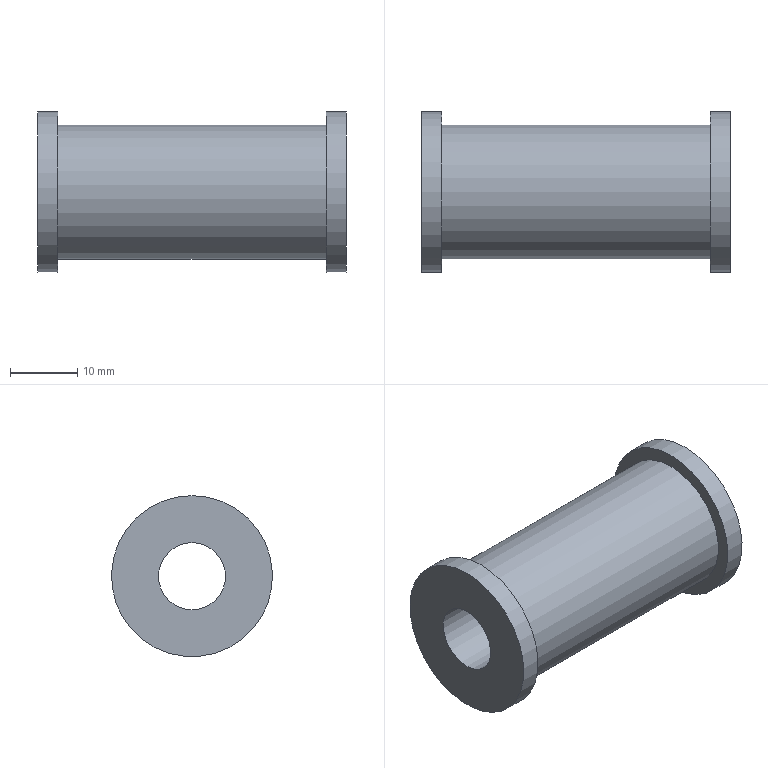Component | NX | JOURNAL_2 | 1 solid | 8 faces | box 46 x 24 x 24 mm | volume 11668 mm3 | plane 4 | cylinder 4 | commonest cylinder face diameters 24 x2 10 x1 20 x1
STEP:
#1=CARTESIAN_POINT('',(0.,0.,0.));
#2=DIRECTION('',(0.,0.,1.));
#3=DIRECTION('',(1.,0.,0.));
#4=AXIS2_PLACEMENT_3D('',#1,#2,#3);
#5=CARTESIAN_POINT('',(14.,-185.74,330.752));
#6=VERTEX_POINT('',#5);
#7=CARTESIAN_POINT('',(14.,-185.74,325.752));
#8=DIRECTION('',(-1.,0.,0.));
#9=DIRECTION('',(0.,0.,1.));
#10=AXIS2_PLACEMENT_3D('',#7,#8,#9);
#11=CIRCLE('',#10,5.);
#12=CARTESIAN_POINT('',(14.,-185.74,313.752));
#13=DIRECTION('',(1.,0.,0.));
#14=DIRECTION('',(0.,0.,-1.));
#15=AXIS2_PLACEMENT_3D('',#12,#13,#14);
#16=PLANE('',#15);
#17=CARTESIAN_POINT('',(-17.,0.));
#18=CARTESIAN_POINT('',(-17.,8.66));
#19=CARTESIAN_POINT('',(-9.5,4.33));
#20=CARTESIAN_POINT('',(-2.,0.));
#21=CARTESIAN_POINT('',(-9.5,-4.33));
#22=CARTESIAN_POINT('',(-17.,-8.66));
#23=CARTESIAN_POINT('',(-17.,0.));
#24=(BOUNDED_CURVE()B_SPLINE_CURVE(2,(#17,#18,#19,#20,#21,#22,#23),.UNSPECIFIED.,.T.,.F.)B_SPLINE_CURVE_WITH_KNOTS((1,2,2,2,2,1),(-2.094,0.,2.094,4.189,6.283,8.378),.UNSPECIFIED.)CURVE()GEOMETRIC_REPRESENTATION_ITEM()RATIONAL_B_SPLINE_CURVE((1.,0.5,1.,0.5,1.,0.5,1.))REPRESENTATION_ITEM(''));
#25=(GEOMETRIC_REPRESENTATION_CONTEXT(2)PARAMETRIC_REPRESENTATION_CONTEXT()REPRESENTATION_CONTEXT('',''));
#26=DEFINITIONAL_REPRESENTATION('',(#24),#25);
#27=PCURVE('',#16,#26);
#28=CARTESIAN_POINT('',(-32.,-185.74,325.752));
#29=DIRECTION('',(-1.,0.,0.));
#30=DIRECTION('',(0.,0.,1.));
#31=AXIS2_PLACEMENT_3D('',#28,#29,#30);
#32=CYLINDRICAL_SURFACE('',#31,5.);
#33=CARTESIAN_POINT('',(0.,-46.));
#34=DIRECTION('',(1.,0.));
#35=VECTOR('',#34,1.);
#36=LINE('',#33,#35);
#37=(GEOMETRIC_REPRESENTATION_CONTEXT(2)PARAMETRIC_REPRESENTATION_CONTEXT()REPRESENTATION_CONTEXT('',''));
#38=DEFINITIONAL_REPRESENTATION('',(#36),#37);
#39=PCURVE('',#32,#38);
#40=SURFACE_CURVE('',#11,(#27,#39),.PCURVE_S1.);
#41=EDGE_CURVE('',#6,#6,#40,.T.);
#42=ORIENTED_EDGE('',*,*,#41,.T.);
#43=EDGE_LOOP('',(#42));
#44=FACE_BOUND('',#43,.T.);
#45=CARTESIAN_POINT('',(14.,-185.74,337.752));
#46=VERTEX_POINT('',#45);
#47=CARTESIAN_POINT('',(14.,-185.74,325.752));
#48=DIRECTION('',(-1.,0.,0.));
#49=DIRECTION('',(0.,0.,1.));
#50=AXIS2_PLACEMENT_3D('',#47,#48,#49);
#51=CIRCLE('',#50,12.);
#52=CARTESIAN_POINT('',(-24.,0.));
#53=CARTESIAN_POINT('',(-24.,20.785));
#54=CARTESIAN_POINT('',(-6.,10.392));
#55=CARTESIAN_POINT('',(12.,0.));
#56=CARTESIAN_POINT('',(-6.,-10.392));
#57=CARTESIAN_POINT('',(-24.,-20.785));
#58=CARTESIAN_POINT('',(-24.,0.));
#59=(BOUNDED_CURVE()B_SPLINE_CURVE(2,(#52,#53,#54,#55,#56,#57,#58),.UNSPECIFIED.,.T.,.F.)B_SPLINE_CURVE_WITH_KNOTS((1,2,2,2,2,1),(-2.094,0.,2.094,4.189,6.283,8.378),.UNSPECIFIED.)CURVE()GEOMETRIC_REPRESENTATION_ITEM()RATIONAL_B_SPLINE_CURVE((1.,0.5,1.,0.5,1.,0.5,1.))REPRESENTATION_ITEM(''));
#60=(GEOMETRIC_REPRESENTATION_CONTEXT(2)PARAMETRIC_REPRESENTATION_CONTEXT()REPRESENTATION_CONTEXT('',''));
#61=DEFINITIONAL_REPRESENTATION('',(#59),#60);
#62=PCURVE('',#16,#61);
#63=CARTESIAN_POINT('',(-32.,-185.74,325.752));
#64=DIRECTION('',(-1.,0.,0.));
#65=DIRECTION('',(0.,0.,1.));
#66=AXIS2_PLACEMENT_3D('',#63,#64,#65);
#67=CYLINDRICAL_SURFACE('',#66,12.);
#68=CARTESIAN_POINT('',(0.,-46.));
#69=DIRECTION('',(1.,0.));
#70=VECTOR('',#69,1.);
#71=LINE('',#68,#70);
#72=(GEOMETRIC_REPRESENTATION_CONTEXT(2)PARAMETRIC_REPRESENTATION_CONTEXT()REPRESENTATION_CONTEXT('',''));
#73=DEFINITIONAL_REPRESENTATION('',(#71),#72);
#74=PCURVE('',#67,#73);
#75=SURFACE_CURVE('',#51,(#62,#74),.PCURVE_S1.);
#76=EDGE_CURVE('',#46,#46,#75,.T.);
#77=ORIENTED_EDGE('',*,*,#76,.F.);
#78=EDGE_LOOP('',(#77));
#79=FACE_BOUND('',#78,.T.);
#80=ADVANCED_FACE('',(#44,#79),#16,.T.);
#81=CARTESIAN_POINT('',(-32.,-185.74,330.752));
#82=VERTEX_POINT('',#81);
#83=CARTESIAN_POINT('',(-32.,-185.74,325.752));
#84=DIRECTION('',(-1.,0.,0.));
#85=DIRECTION('',(0.,0.,1.));
#86=AXIS2_PLACEMENT_3D('',#83,#84,#85);
#87=CIRCLE('',#86,5.);
#88=CARTESIAN_POINT('',(0.,0.));
#89=DIRECTION('',(1.,0.));
#90=VECTOR('',#89,1.);
#91=LINE('',#88,#90);
#92=(GEOMETRIC_REPRESENTATION_CONTEXT(2)PARAMETRIC_REPRESENTATION_CONTEXT()REPRESENTATION_CONTEXT('',''));
#93=DEFINITIONAL_REPRESENTATION('',(#91),#92);
#94=PCURVE('',#32,#93);
#95=CARTESIAN_POINT('',(-32.,-185.74,320.752));
#96=DIRECTION('',(-1.,0.,0.));
#97=DIRECTION('',(0.,0.,1.));
#98=AXIS2_PLACEMENT_3D('',#95,#96,#97);
#99=PLANE('',#98);
#100=CARTESIAN_POINT('',(5.,0.));
#101=DIRECTION('',(1.,0.));
#102=AXIS2_PLACEMENT_2D('',#100,#101);
#103=CIRCLE('',#102,5.);
#104=(GEOMETRIC_REPRESENTATION_CONTEXT(2)PARAMETRIC_REPRESENTATION_CONTEXT()REPRESENTATION_CONTEXT('',''));
#105=DEFINITIONAL_REPRESENTATION('',(#103),#104);
#106=PCURVE('',#99,#105);
#107=SURFACE_CURVE('',#87,(#94,#106),.PCURVE_S1.);
#108=EDGE_CURVE('',#82,#82,#107,.T.);
#109=ORIENTED_EDGE('',*,*,#108,.F.);
#110=CARTESIAN_POINT('',(14.,-185.74,330.752));
#111=CARTESIAN_POINT('',(-32.,-185.74,330.752));
#112=B_SPLINE_CURVE_WITH_KNOTS('',1,(#110,#111),.UNSPECIFIED.,.F.,.F.,(2,2),(-46.,0.),.PIECEWISE_BEZIER_KNOTS.);
#113=CARTESIAN_POINT('',(0.,0.));
#114=DIRECTION('',(0.,1.));
#115=VECTOR('',#114,1.);
#116=LINE('',#113,#115);
#117=(GEOMETRIC_REPRESENTATION_CONTEXT(2)PARAMETRIC_REPRESENTATION_CONTEXT()REPRESENTATION_CONTEXT('',''));
#118=DEFINITIONAL_REPRESENTATION('',(#116),#117);
#119=PCURVE('',#32,#118);
#120=CARTESIAN_POINT('',(6.283,0.));
#121=DIRECTION('',(0.,1.));
#122=VECTOR('',#121,1.);
#123=LINE('',#120,#122);
#124=(GEOMETRIC_REPRESENTATION_CONTEXT(2)PARAMETRIC_REPRESENTATION_CONTEXT()REPRESENTATION_CONTEXT('',''));
#125=DEFINITIONAL_REPRESENTATION('',(#123),#124);
#126=PCURVE('',#32,#125);
#127=SEAM_CURVE('',#112,(#119,#126),.PCURVE_S1.);
#128=EDGE_CURVE('',#6,#82,#127,.T.);
#129=ORIENTED_EDGE('',*,*,#128,.F.);
#130=ORIENTED_EDGE('',*,*,#41,.T.);
#131=ORIENTED_EDGE('',*,*,#128,.T.);
#132=EDGE_LOOP('',(#109,#129,#130,#131));
#133=FACE_BOUND('',#132,.F.);
#134=ADVANCED_FACE('',(#133),#32,.F.);
#135=CARTESIAN_POINT('',(-32.,-185.74,337.752));
#136=VERTEX_POINT('',#135);
#137=CARTESIAN_POINT('',(-32.,-185.74,325.752));
#138=DIRECTION('',(-1.,0.,0.));
#139=DIRECTION('',(0.,0.,1.));
#140=AXIS2_PLACEMENT_3D('',#137,#138,#139);
#141=CIRCLE('',#140,12.);
#142=CARTESIAN_POINT('',(5.,0.));
#143=DIRECTION('',(1.,0.));
#144=AXIS2_PLACEMENT_2D('',#142,#143);
#145=CIRCLE('',#144,12.);
#146=(GEOMETRIC_REPRESENTATION_CONTEXT(2)PARAMETRIC_REPRESENTATION_CONTEXT()REPRESENTATION_CONTEXT('',''));
#147=DEFINITIONAL_REPRESENTATION('',(#145),#146);
#148=PCURVE('',#99,#147);
#149=CARTESIAN_POINT('',(-32.,-185.74,325.752));
#150=DIRECTION('',(-1.,0.,0.));
#151=DIRECTION('',(0.,0.,1.));
#152=AXIS2_PLACEMENT_3D('',#149,#150,#151);
#153=CYLINDRICAL_SURFACE('',#152,12.);
#154=CARTESIAN_POINT('',(0.,0.));
#155=DIRECTION('',(1.,0.));
#156=VECTOR('',#155,1.);
#157=LINE('',#154,#156);
#158=(GEOMETRIC_REPRESENTATION_CONTEXT(2)PARAMETRIC_REPRESENTATION_CONTEXT()REPRESENTATION_CONTEXT('',''));
#159=DEFINITIONAL_REPRESENTATION('',(#157),#158);
#160=PCURVE('',#153,#159);
#161=SURFACE_CURVE('',#141,(#148,#160),.PCURVE_S1.);
#162=EDGE_CURVE('',#136,#136,#161,.T.);
#163=ORIENTED_EDGE('',*,*,#162,.T.);
#164=EDGE_LOOP('',(#163));
#165=FACE_BOUND('',#164,.T.);
#166=ORIENTED_EDGE('',*,*,#108,.F.);
#167=EDGE_LOOP('',(#166));
#168=FACE_BOUND('',#167,.T.);
#169=ADVANCED_FACE('',(#165,#168),#99,.T.);
#170=CARTESIAN_POINT('',(-29.,-185.74,337.752));
#171=VERTEX_POINT('',#170);
#172=CARTESIAN_POINT('',(-29.,-185.74,325.752));
#173=DIRECTION('',(-1.,0.,0.));
#174=DIRECTION('',(0.,0.,1.));
#175=AXIS2_PLACEMENT_3D('',#172,#173,#174);
#176=CIRCLE('',#175,12.);
#177=CARTESIAN_POINT('',(0.,-3.));
#178=DIRECTION('',(1.,0.));
#179=VECTOR('',#178,1.);
#180=LINE('',#177,#179);
#181=(GEOMETRIC_REPRESENTATION_CONTEXT(2)PARAMETRIC_REPRESENTATION_CONTEXT()REPRESENTATION_CONTEXT('',''));
#182=DEFINITIONAL_REPRESENTATION('',(#180),#181);
#183=PCURVE('',#153,#182);
#184=CARTESIAN_POINT('',(-29.,-185.74,313.752));
#185=DIRECTION('',(1.,0.,0.));
#186=DIRECTION('',(0.,0.,-1.));
#187=AXIS2_PLACEMENT_3D('',#184,#185,#186);
#188=PLANE('',#187);
#189=CARTESIAN_POINT('',(-24.,0.));
#190=CARTESIAN_POINT('',(-24.,20.785));
#191=CARTESIAN_POINT('',(-6.,10.392));
#192=CARTESIAN_POINT('',(12.,0.));
#193=CARTESIAN_POINT('',(-6.,-10.392));
#194=CARTESIAN_POINT('',(-24.,-20.785));
#195=CARTESIAN_POINT('',(-24.,0.));
#196=(BOUNDED_CURVE()B_SPLINE_CURVE(2,(#189,#190,#191,#192,#193,#194,#195),.UNSPECIFIED.,.T.,.F.)B_SPLINE_CURVE_WITH_KNOTS((1,2,2,2,2,1),(-2.094,0.,2.094,4.189,6.283,8.378),.UNSPECIFIED.)CURVE()GEOMETRIC_REPRESENTATION_ITEM()RATIONAL_B_SPLINE_CURVE((1.,0.5,1.,0.5,1.,0.5,1.))REPRESENTATION_ITEM(''));
#197=(GEOMETRIC_REPRESENTATION_CONTEXT(2)PARAMETRIC_REPRESENTATION_CONTEXT()REPRESENTATION_CONTEXT('',''));
#198=DEFINITIONAL_REPRESENTATION('',(#196),#197);
#199=PCURVE('',#188,#198);
#200=SURFACE_CURVE('',#176,(#183,#199),.PCURVE_S1.);
#201=EDGE_CURVE('',#171,#171,#200,.T.);
#202=ORIENTED_EDGE('',*,*,#201,.T.);
#203=CARTESIAN_POINT('',(-29.,-185.74,337.752));
#204=CARTESIAN_POINT('',(-32.,-185.74,337.752));
#205=B_SPLINE_CURVE_WITH_KNOTS('',1,(#203,#204),.UNSPECIFIED.,.F.,.F.,(2,2),(-3.,0.),.PIECEWISE_BEZIER_KNOTS.);
#206=CARTESIAN_POINT('',(6.283,0.));
#207=DIRECTION('',(0.,1.));
#208=VECTOR('',#207,1.);
#209=LINE('',#206,#208);
#210=(GEOMETRIC_REPRESENTATION_CONTEXT(2)PARAMETRIC_REPRESENTATION_CONTEXT()REPRESENTATION_CONTEXT('',''));
#211=DEFINITIONAL_REPRESENTATION('',(#209),#210);
#212=PCURVE('',#153,#211);
#213=CARTESIAN_POINT('',(0.,0.));
#214=DIRECTION('',(0.,1.));
#215=VECTOR('',#214,1.);
#216=LINE('',#213,#215);
#217=(GEOMETRIC_REPRESENTATION_CONTEXT(2)PARAMETRIC_REPRESENTATION_CONTEXT()REPRESENTATION_CONTEXT('',''));
#218=DEFINITIONAL_REPRESENTATION('',(#216),#217);
#219=PCURVE('',#153,#218);
#220=SEAM_CURVE('',#205,(#212,#219),.PCURVE_S1.);
#221=EDGE_CURVE('',#171,#136,#220,.T.);
#222=ORIENTED_EDGE('',*,*,#221,.T.);
#223=ORIENTED_EDGE('',*,*,#162,.F.);
#224=ORIENTED_EDGE('',*,*,#221,.F.);
#225=EDGE_LOOP('',(#202,#222,#223,#224));
#226=FACE_BOUND('',#225,.T.);
#227=ADVANCED_FACE('',(#226),#153,.T.);
#228=CARTESIAN_POINT('',(-29.,-185.74,335.752));
#229=VERTEX_POINT('',#228);
#230=CARTESIAN_POINT('',(-29.,-185.74,325.752));
#231=DIRECTION('',(-1.,0.,0.));
#232=DIRECTION('',(0.,0.,1.));
#233=AXIS2_PLACEMENT_3D('',#230,#231,#232);
#234=CIRCLE('',#233,10.);
#235=CARTESIAN_POINT('',(-22.,0.));
#236=CARTESIAN_POINT('',(-22.,17.321));
#237=CARTESIAN_POINT('',(-7.,8.66));
#238=CARTESIAN_POINT('',(8.,0.));
#239=CARTESIAN_POINT('',(-7.,-8.66));
#240=CARTESIAN_POINT('',(-22.,-17.321));
#241=CARTESIAN_POINT('',(-22.,0.));
#242=(BOUNDED_CURVE()B_SPLINE_CURVE(2,(#235,#236,#237,#238,#239,#240,#241),.UNSPECIFIED.,.T.,.F.)B_SPLINE_CURVE_WITH_KNOTS((1,2,2,2,2,1),(-2.094,0.,2.094,4.189,6.283,8.378),.UNSPECIFIED.)CURVE()GEOMETRIC_REPRESENTATION_ITEM()RATIONAL_B_SPLINE_CURVE((1.,0.5,1.,0.5,1.,0.5,1.))REPRESENTATION_ITEM(''));
#243=(GEOMETRIC_REPRESENTATION_CONTEXT(2)PARAMETRIC_REPRESENTATION_CONTEXT()REPRESENTATION_CONTEXT('',''));
#244=DEFINITIONAL_REPRESENTATION('',(#242),#243);
#245=PCURVE('',#188,#244);
#246=CARTESIAN_POINT('',(-32.,-185.74,325.752));
#247=DIRECTION('',(-1.,0.,0.));
#248=DIRECTION('',(0.,0.,1.));
#249=AXIS2_PLACEMENT_3D('',#246,#247,#248);
#250=CYLINDRICAL_SURFACE('',#249,10.);
#251=CARTESIAN_POINT('',(0.,-3.));
#252=DIRECTION('',(1.,0.));
#253=VECTOR('',#252,1.);
#254=LINE('',#251,#253);
#255=(GEOMETRIC_REPRESENTATION_CONTEXT(2)PARAMETRIC_REPRESENTATION_CONTEXT()REPRESENTATION_CONTEXT('',''));
#256=DEFINITIONAL_REPRESENTATION('',(#254),#255);
#257=PCURVE('',#250,#256);
#258=SURFACE_CURVE('',#234,(#245,#257),.PCURVE_S1.);
#259=EDGE_CURVE('',#229,#229,#258,.T.);
#260=ORIENTED_EDGE('',*,*,#259,.T.);
#261=EDGE_LOOP('',(#260));
#262=FACE_BOUND('',#261,.T.);
#263=ORIENTED_EDGE('',*,*,#201,.F.);
#264=EDGE_LOOP('',(#263));
#265=FACE_BOUND('',#264,.T.);
#266=ADVANCED_FACE('',(#262,#265),#188,.T.);
#267=CARTESIAN_POINT('',(11.,-185.74,335.752));
#268=VERTEX_POINT('',#267);
#269=CARTESIAN_POINT('',(11.,-185.74,325.752));
#270=DIRECTION('',(-1.,0.,0.));
#271=DIRECTION('',(0.,0.,1.));
#272=AXIS2_PLACEMENT_3D('',#269,#270,#271);
#273=CIRCLE('',#272,10.);
#274=CARTESIAN_POINT('',(0.,-43.));
#275=DIRECTION('',(1.,0.));
#276=VECTOR('',#275,1.);
#277=LINE('',#274,#276);
#278=(GEOMETRIC_REPRESENTATION_CONTEXT(2)PARAMETRIC_REPRESENTATION_CONTEXT()REPRESENTATION_CONTEXT('',''));
#279=DEFINITIONAL_REPRESENTATION('',(#277),#278);
#280=PCURVE('',#250,#279);
#281=CARTESIAN_POINT('',(11.,-185.74,315.752));
#282=DIRECTION('',(-1.,0.,0.));
#283=DIRECTION('',(0.,0.,1.));
#284=AXIS2_PLACEMENT_3D('',#281,#282,#283);
#285=PLANE('',#284);
#286=CARTESIAN_POINT('',(10.,0.));
#287=DIRECTION('',(1.,0.));
#288=AXIS2_PLACEMENT_2D('',#286,#287);
#289=CIRCLE('',#288,10.);
#290=(GEOMETRIC_REPRESENTATION_CONTEXT(2)PARAMETRIC_REPRESENTATION_CONTEXT()REPRESENTATION_CONTEXT('',''));
#291=DEFINITIONAL_REPRESENTATION('',(#289),#290);
#292=PCURVE('',#285,#291);
#293=SURFACE_CURVE('',#273,(#280,#292),.PCURVE_S1.);
#294=EDGE_CURVE('',#268,#268,#293,.T.);
#295=ORIENTED_EDGE('',*,*,#294,.T.);
#296=CARTESIAN_POINT('',(11.,-185.74,335.752));
#297=CARTESIAN_POINT('',(-29.,-185.74,335.752));
#298=B_SPLINE_CURVE_WITH_KNOTS('',1,(#296,#297),.UNSPECIFIED.,.F.,.F.,(2,2),(-43.,-3.),.PIECEWISE_BEZIER_KNOTS.);
#299=CARTESIAN_POINT('',(6.283,0.));
#300=DIRECTION('',(0.,1.));
#301=VECTOR('',#300,1.);
#302=LINE('',#299,#301);
#303=(GEOMETRIC_REPRESENTATION_CONTEXT(2)PARAMETRIC_REPRESENTATION_CONTEXT()REPRESENTATION_CONTEXT('',''));
#304=DEFINITIONAL_REPRESENTATION('',(#302),#303);
#305=PCURVE('',#250,#304);
#306=CARTESIAN_POINT('',(0.,0.));
#307=DIRECTION('',(0.,1.));
#308=VECTOR('',#307,1.);
#309=LINE('',#306,#308);
#310=(GEOMETRIC_REPRESENTATION_CONTEXT(2)PARAMETRIC_REPRESENTATION_CONTEXT()REPRESENTATION_CONTEXT('',''));
#311=DEFINITIONAL_REPRESENTATION('',(#309),#310);
#312=PCURVE('',#250,#311);
#313=SEAM_CURVE('',#298,(#305,#312),.PCURVE_S1.);
#314=EDGE_CURVE('',#268,#229,#313,.T.);
#315=ORIENTED_EDGE('',*,*,#314,.T.);
#316=ORIENTED_EDGE('',*,*,#259,.F.);
#317=ORIENTED_EDGE('',*,*,#314,.F.);
#318=EDGE_LOOP('',(#295,#315,#316,#317));
#319=FACE_BOUND('',#318,.T.);
#320=ADVANCED_FACE('',(#319),#250,.T.);
#321=CARTESIAN_POINT('',(11.,-185.74,337.752));
#322=VERTEX_POINT('',#321);
#323=CARTESIAN_POINT('',(11.,-185.74,325.752));
#324=DIRECTION('',(-1.,0.,0.));
#325=DIRECTION('',(0.,0.,1.));
#326=AXIS2_PLACEMENT_3D('',#323,#324,#325);
#327=CIRCLE('',#326,12.);
#328=CARTESIAN_POINT('',(10.,0.));
#329=DIRECTION('',(1.,0.));
#330=AXIS2_PLACEMENT_2D('',#328,#329);
#331=CIRCLE('',#330,12.);
#332=(GEOMETRIC_REPRESENTATION_CONTEXT(2)PARAMETRIC_REPRESENTATION_CONTEXT()REPRESENTATION_CONTEXT('',''));
#333=DEFINITIONAL_REPRESENTATION('',(#331),#332);
#334=PCURVE('',#285,#333);
#335=CARTESIAN_POINT('',(0.,-43.));
#336=DIRECTION('',(1.,0.));
#337=VECTOR('',#336,1.);
#338=LINE('',#335,#337);
#339=(GEOMETRIC_REPRESENTATION_CONTEXT(2)PARAMETRIC_REPRESENTATION_CONTEXT()REPRESENTATION_CONTEXT('',''));
#340=DEFINITIONAL_REPRESENTATION('',(#338),#339);
#341=PCURVE('',#67,#340);
#342=SURFACE_CURVE('',#327,(#334,#341),.PCURVE_S1.);
#343=EDGE_CURVE('',#322,#322,#342,.T.);
#344=ORIENTED_EDGE('',*,*,#343,.T.);
#345=EDGE_LOOP('',(#344));
#346=FACE_BOUND('',#345,.T.);
#347=ORIENTED_EDGE('',*,*,#294,.F.);
#348=EDGE_LOOP('',(#347));
#349=FACE_BOUND('',#348,.T.);
#350=ADVANCED_FACE('',(#346,#349),#285,.T.);
#351=ORIENTED_EDGE('',*,*,#76,.T.);
#352=CARTESIAN_POINT('',(14.,-185.74,337.752));
#353=CARTESIAN_POINT('',(11.,-185.74,337.752));
#354=B_SPLINE_CURVE_WITH_KNOTS('',1,(#352,#353),.UNSPECIFIED.,.F.,.F.,(2,2),(-46.,-43.),.PIECEWISE_BEZIER_KNOTS.);
#355=CARTESIAN_POINT('',(6.283,0.));
#356=DIRECTION('',(0.,1.));
#357=VECTOR('',#356,1.);
#358=LINE('',#355,#357);
#359=(GEOMETRIC_REPRESENTATION_CONTEXT(2)PARAMETRIC_REPRESENTATION_CONTEXT()REPRESENTATION_CONTEXT('',''));
#360=DEFINITIONAL_REPRESENTATION('',(#358),#359);
#361=PCURVE('',#67,#360);
#362=CARTESIAN_POINT('',(0.,0.));
#363=DIRECTION('',(0.,1.));
#364=VECTOR('',#363,1.);
#365=LINE('',#362,#364);
#366=(GEOMETRIC_REPRESENTATION_CONTEXT(2)PARAMETRIC_REPRESENTATION_CONTEXT()REPRESENTATION_CONTEXT('',''));
#367=DEFINITIONAL_REPRESENTATION('',(#365),#366);
#368=PCURVE('',#67,#367);
#369=SEAM_CURVE('',#354,(#361,#368),.PCURVE_S1.);
#370=EDGE_CURVE('',#46,#322,#369,.T.);
#371=ORIENTED_EDGE('',*,*,#370,.T.);
#372=ORIENTED_EDGE('',*,*,#343,.F.);
#373=ORIENTED_EDGE('',*,*,#370,.F.);
#374=EDGE_LOOP('',(#351,#371,#372,#373));
#375=FACE_BOUND('',#374,.T.);
#376=ADVANCED_FACE('',(#375),#67,.T.);
#377=CLOSED_SHELL('',(#80,#134,#169,#227,#266,#320,#350,#376));
#378=MANIFOLD_SOLID_BREP('',#377);
#379=(LENGTH_UNIT()NAMED_UNIT(*)SI_UNIT(.MILLI.,.METRE.));
#380=UNCERTAINTY_MEASURE_WITH_UNIT(LENGTH_MEASURE(0.00001),#379,'','');
#381=(NAMED_UNIT(*)PLANE_ANGLE_UNIT()SI_UNIT($,.RADIAN.));
#382=(NAMED_UNIT(*)SI_UNIT($,.STERADIAN.)SOLID_ANGLE_UNIT());
#383=(GEOMETRIC_REPRESENTATION_CONTEXT(3)GLOBAL_UNCERTAINTY_ASSIGNED_CONTEXT((#380))GLOBAL_UNIT_ASSIGNED_CONTEXT((#379,#381,#382))REPRESENTATION_CONTEXT('',''));
#384=ADVANCED_BREP_SHAPE_REPRESENTATION('',(#4,#378),#383);